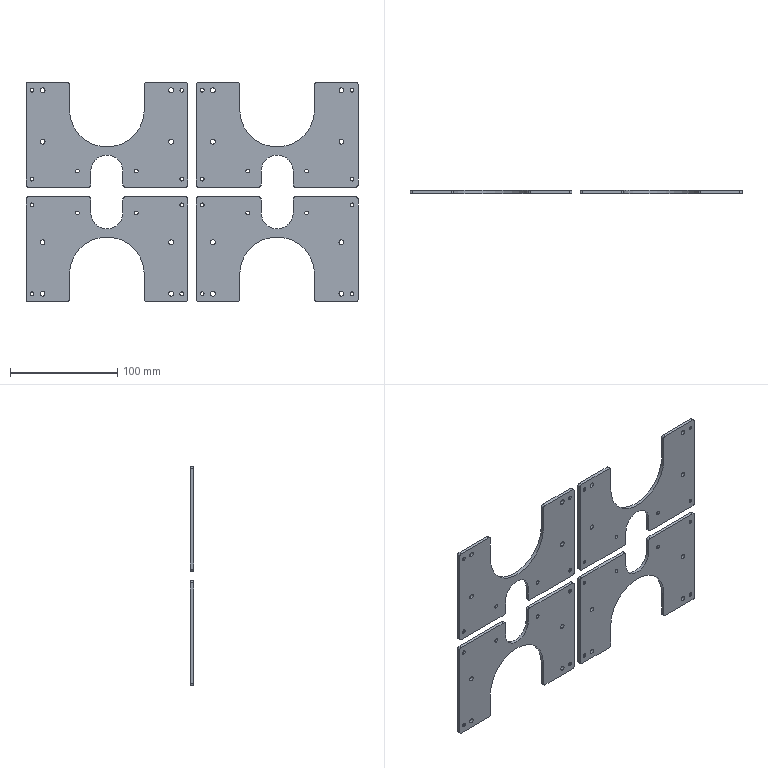CAM job | Mastercam | mm | 4 operations | part box 310 x 3 x 205
1. Contour (Ramp) | 3 - 3 倒角刀
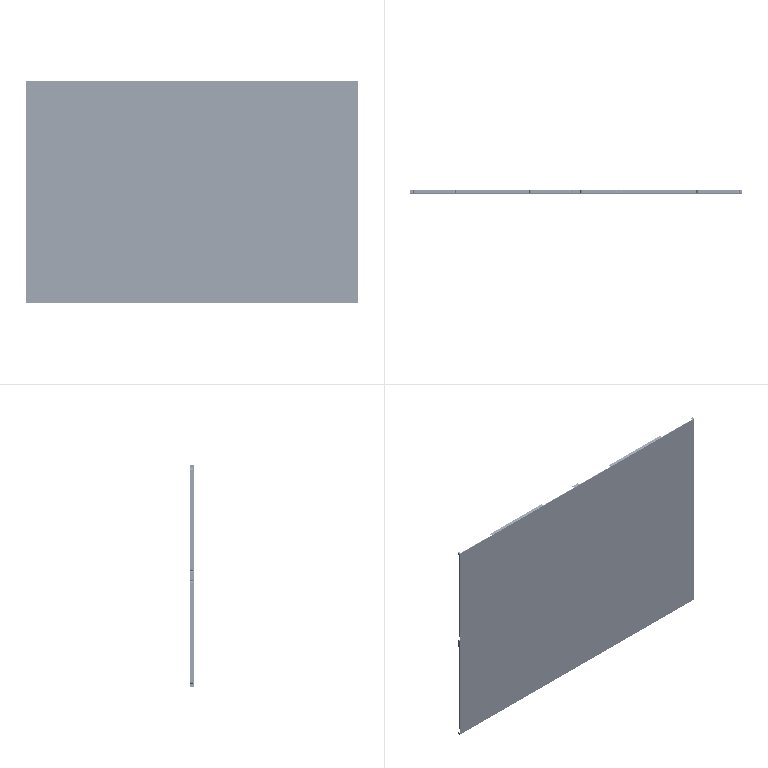2. Drill/Counterbore | 7 - 4 倒角刀
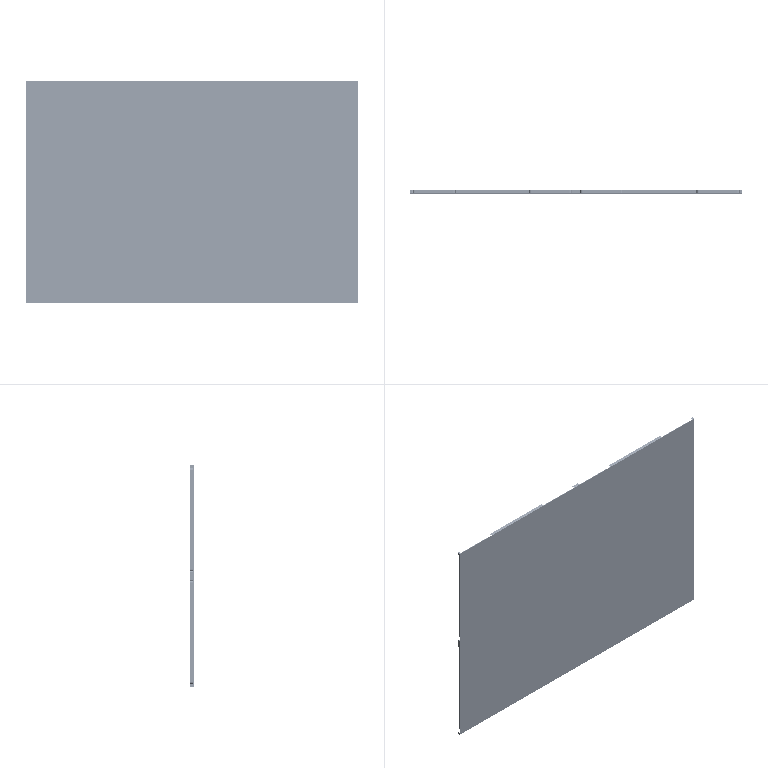3. Contour (2D chamfer) | 7 - 4 倒角刀
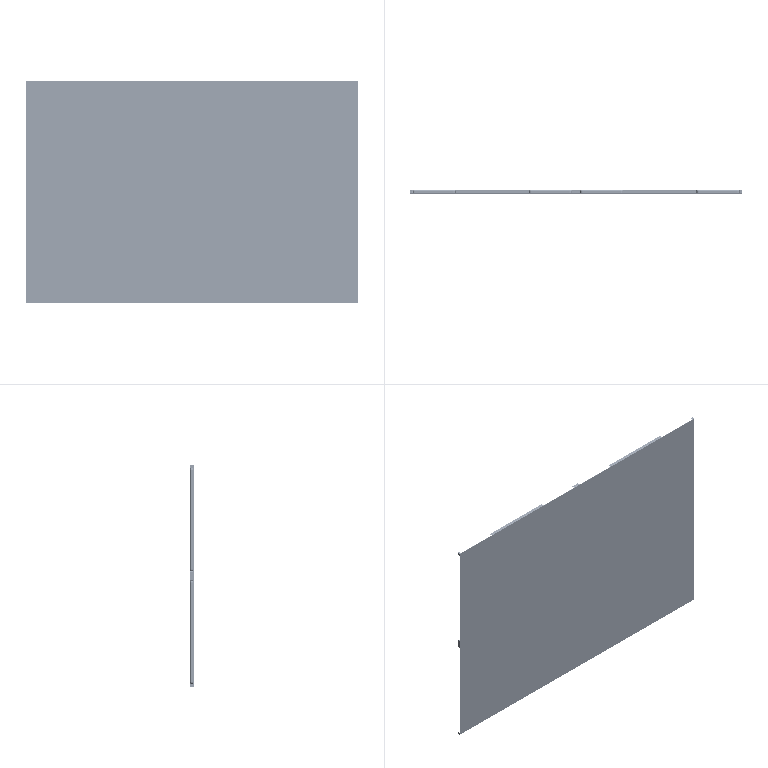4. Contour (Ramp) | 2 - 2 平铣刀